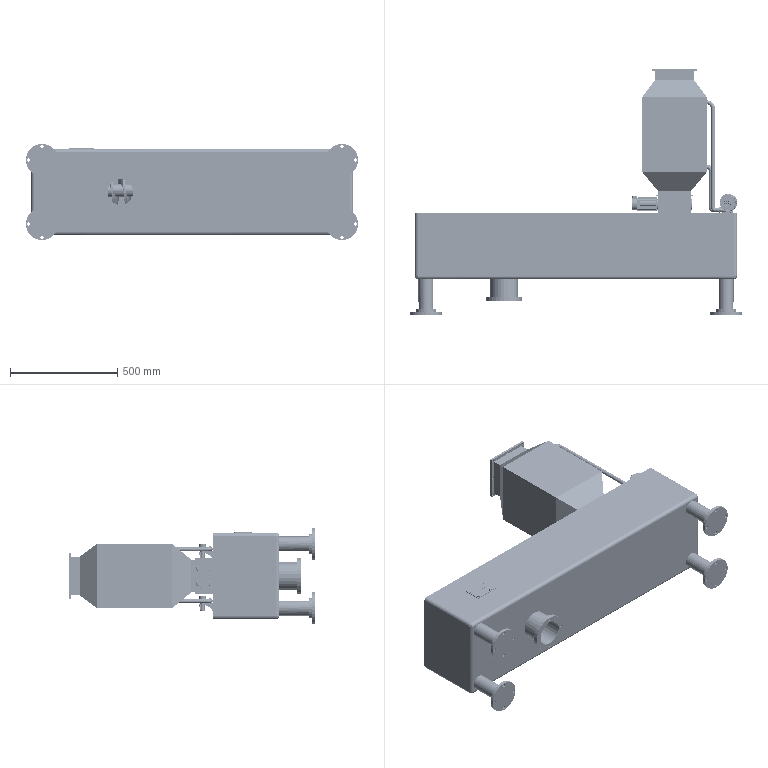Assembly | SolidWorks | mm | 45 component files | 49 solids | 6912 faces | box 1548.53 x 1145.2 x 448.53 mm | volume 120941884 mm3 | plane 3366 | cylinder 2732 | torus 522 | spline 126 | sphere 114 | cone 52 | commonest cylinder face diameters 0.75 x556 0.3 x432 15 x252 17 x208 6 x112 1.5 x64 10 x52 12.958 x45
Bill of materials:
90ST-M02430 | 2 |  | Motor-like body shaped as a long square-section housing. One end has a square mounting flange with four corner through-holes and a single cylindrical shaft. The other end has a short cylindrical rear cap with a small boxy protrusion on its side.
CrushingCutterBar | 2 |  | Solid straight cylindrical rod with a thin, slightly larger-diameter disc head at one end (pin- or rivet-like shape).
CrushingCutterDisc | 9 |  | Thick disc with a central round bore that has one rectangular keyway, and four curved, hook-shaped teeth evenly spaced around the rim and all curving the same way.
EndCover | 2 |  | Solid stepped disc: a larger-diameter disc joined coaxially to a thinner, smaller-diameter disc or boss on one face.
Fan | 2 |  | Assembly-like body that appears to be a centrifugal blower: a spiral (volute) housing with a tangential round outlet ending in a flange, a cylindrical housing on top with a perforated circular vent pattern, a finned cylindrical body and end cap below, a side box, and a plate bracket with mounting holes.
FeedBox | 1 |  | Rectangular box-shaped duct section with pyramidal tapers at both ends, each ending in a smaller rectangular neck with a bolted flange.
HeatPipe | 8 |  | Hollow round tube bent in one plane into a serpentine shape: six parallel straight runs joined by sharp, mitred-looking 180-degree returns, with both open ends on the same side.
PlateOne | 1 |  | Flat rectangular plate of uniform thickness with two round through-holes at diagonally opposite corners.
PlateTwo | 1 |  | Plain flat rectangular plate of uniform thickness with no visible holes or features.
Housing | 1 |  | Long rectangular box with lightly rounded edges. One long face carries four cylindrical stub pegs near its ends and a short round nozzle with a flange and small bolt holes. A small square opening is cut in the top face.
IMB3H56-90GeneralMotor[YS-561-4-B3] | 1 |  | Motor-like body shaped as a horizontal cylindrical housing. It has fins running along its length, bolt-down mounting feet with holes, and a rectangular box on top. A rounded cap covers one end. A small cylindrical shaft sticks out from the middle of the other end.
MotorEndCover | 2 |  | Stepped annular disc: a flat ring with a raised, smaller-diameter boss on one face and a central round bore with one rectangular keyway.
PipeOne | 1 |  | Hollow round tube with a long straight middle section and a short 90-degree bent leg at each end, the two legs pointing in opposite directions in one plane (Z or offset shape).
PipeTwo | 1 |  | Long, slender hollow round tube with small 90-degree bends at both ends turning in opposite directions in one plane (Z or offset shape). The close-up shows a chamfered end edge.
Screen | 1 |  | Thin rectangular plate with rounded corners. The top face has several low raised features, and a slightly smaller, thicker block sits under the plate.
SpiralConveyorRod | 1 |  | Straight cylindrical shaft with a continuous thin helical flight wrapped along its length. The shaft sticks out a short way past the flight at the end.
SupportFrame | 2 |  | Bent thin-plate bracket. A rectangular main face has two large round through-holes. A narrow side flange has three small holes, and there is a short return lip on the opposite edge.
SupportFrameA | 2 |  | Shallow U-shaped channel or cover made from thin plate: a flat rectangular top with two short downturned side flanges. One flange has three round holes.
SupportLeg | 4 |  | Flat circular disc with a large central through-bore and four smaller holes evenly spaced on a bolt circle. A raised hub of smaller diameter, concentric with the disc, sits on one face.
TopCover | 1 |  | Long, thin rectangular panel with rounded corners. It has one square through-cutout with small holes around its edge, and several thin rib or strip features running across the panel on one face.
Mates:
1. concentric | Housing-1 face at (-699.263, -180, 149.263) dir (0, 1, 0) r 35 | SupportLeg-2 face at (-699.263, -165, 149.263) dir (0, -1, 0) r 35
2. coincident | Housing-1 face at (-699.263, -180, 149.263) dir (0, -1, 0) | SupportLeg-2 face at (-699.263, -180, 149.263) dir (0, -1, 0)
3. coincident | Housing-1 face at (0, 0, 200) dir (0, 0, 1) | TopCover-1 face at (-734.95, 285, 200) dir (0, 0, 1)
4. coincident | Housing-1 face at (-750, 0, 0) dir (-1, 0, 0) | TopCover-1 face at (-750, 285, -184.95) dir (-1, 0, 0)
5. coincident | Housing-1 face at (-750, 285, -200) dir (0, 1, 0) | TopCover-1 face at (734.95, 285, -184.95) dir (0, -1, 0)
6. concentric | Housing-1 face at (-454, 142.868, 6.9) dir (1, 0, 0) r 30 | SpiralConveyorRod-2 face at (-407, 142.868, 6.9) dir (1, 0, 0) r 30
7. coincident | TopCover-1 face at (734.95, 295, -184.95) dir (0, 1, 0) | SupportFrame-1 face at (384.19, 295, 85) dir (0, -1, 0)
8. coincident | TopCover-1 face at (384.29, 72.868, -75) dir (1, 0, 0) | SupportFrame-1 face at (384.29, 295.1, 85) dir (1, 0, 0)
9. distance | SupportFrame-1 face at (384.19, 311.439, -85) dir (0, 0, -1) | TopCover-1 face at (384.29, 72.868, -75) dir (0, 0, 1)
10. coincident | TopCover-1 face at (534.29, 72.868, -75) dir (-1, 0, 0) | SupportFrame-2 face at (534.29, 295.1, -85) dir (-1, 0, 0)
11. coincident | TopCover-1 face at (734.95, 295, -184.95) dir (0, 1, 0) | SupportFrame-2 face at (534.39, 295, -85) dir (0, -1, 0)
12. distance | SupportFrame-2 face at (534.39, 295.1, -85) dir (0, 0, -1) | TopCover-1 face at (384.29, 72.868, -75) dir (0, 0, 1)
13. coincident | TopCover-1 face at (734.95, 295, -184.95) dir (0, 1, 0) | SupportFrameA-2 face at (384.29, 295, -75.5) dir (0, -1, 0)
14. coincident | TopCover-1 face at (384.29, 72.868, -75) dir (0, 0, 1) | SupportFrameA-2 face at (384.29, 295.5, -75) dir (0, 0, 1)
15. coincident | SupportFrameA-2 face at (534.29, 374.7, -75.5) dir (1, 0, 0) | SupportFrame-2 face at (534.29, 295.1, -85) dir (-1, 0, 0)
16. coincident | TopCover-1 face at (734.95, 295, -184.95) dir (0, 1, 0) | SupportFrameA-3 face at (534.29, 295, 75.5) dir (0, -1, 0)
17. coincident | TopCover-1 face at (384.29, 72.868, 75) dir (0, 0, -1) | SupportFrameA-3 face at (534.29, 295.5, 75) dir (0, 0, -1)
18. coincident | SupportFrame-1 face at (384.29, 295.1, 85) dir (1, 0, 0) | SupportFrameA-3 face at (384.29, 295.5, 75.5) dir (-1, 0, 0)
19. concentric | SpiralConveyorRod-2 edge at (-407, 142.868, 6.9) dir (1, 0, 0) r 30 | IMB3H56-90GeneralMotor[YS-561-4-B3]-2 face at (-410, 142.868, 6.9) dir (-1, 0, 0) r 4.5
20. coincident | Housing-1 face at (-410, 0, 0) dir (-1, 0, 0) | IMB3H56-90GeneralMotor[YS-561-4-B3]-2 face at (-410, 117.868, 6.9) dir (1, 0, 0)
21. concentric | SupportFrame-1 edge at (384.19, 335.1, 35) dir (-1, 0, 0) r 20 | 60-90SeriesServoMotor[60ST-M00630]-1 face at (403.19, 335.1, 35) dir (1, 0, 0) r 6
22. concentric | SupportFrame-1 edge at (384.19, 335.1, -35) dir (-1, 0, 0) r 20 | 60-90SeriesServoMotor[60ST-M00630]-2 face at (403.19, 335.1, -35) dir (1, 0, 0) r 6
23. parallel | TopCover-1 face at (734.95, 295, -184.95) dir (0, 1, 0) | 60-90SeriesServoMotor[60ST-M00630]-1 face at (370.94, 367.35, 62.375) dir (0, 1, 0)
24. parallel | TopCover-1 face at (734.95, 295, -184.95) dir (0, 1, 0) | 60-90SeriesServoMotor[60ST-M00630]-2 face at (370.94, 367.35, -7.625) dir (0, 1, 0)
25. concentric | SupportFrame-1 edge at (384.19, 335.1, 35) dir (-1, 0, 0) r 20 | MotorEndCover-1 face at (386.19, 335.1, 35) dir (1, 0, 0) r 8
26. concentric | SupportFrame-1 edge at (384.19, 335.1, -35) dir (-1, 0, 0) r 20 | MotorEndCover-2 edge at (379.19, 335.1, -35) dir (1, 0, 0) r 8
27. coincident | SupportFrame-1 face at (384.19, 295.1, 85) dir (-1, 0, 0) | MotorEndCover-2 face at (384.19, 335.1, -35) dir (1, 0, 0)
28. coincident | 60-90SeriesServoMotor[60ST-M00630]-1 face at (379.19, 335.1, 35) dir (1, 0, 0) | MotorEndCover-1 face at (379.19, 335.1, 35) dir (-1, 0, 0)
29. coincident | 60-90SeriesServoMotor[60ST-M00630]-2 face at (379.19, 335.1, -35) dir (1, 0, 0) | MotorEndCover-2 face at (379.19, 335.1, -35) dir (-1, 0, 0)
30. concentric | 60-90SeriesServoMotor[60ST-M00630]-2 face at (403.19, 335.1, -35) dir (1, 0, 0) r 6 | CrushingCutterBar-1 face at (529.19, 335.1, -35) dir (-1, 0, 0) r 8
31. coincident | MotorEndCover-2 face at (386.19, 335.1, -35) dir (1, 0, 0) | CrushingCutterBar-1 face at (386.19, 335.1, -35) dir (-1, 0, 0)
32. concentric | SupportFrame-2 edge at (534.39, 335.1, -35) dir (1, 0, 0) r 20 | EndCover-1 edge at (529.39, 335.1, -35) dir (-1, 0, 0) r 14.92
33. coincident | SupportFrame-2 face at (534.39, 295.1, -85) dir (1, 0, 0) | EndCover-1 face at (534.39, 335.1, -35) dir (-1, 0, 0)
34. concentric | 60-90SeriesServoMotor[60ST-M00630]-1 edge at (402.695, 335.1, 35) dir (-1, 0, 0) r 6 | CrushingCutterBar-2 edge at (386.19, 335.1, 35) dir (1, 0, 0) r 8
35. parallel | 60-90SeriesServoMotor[60ST-M00630]-2 face at (384.065, 342.6, -35) dir (0, 1, 0) | CrushingCutterBar-1 face at (529.19, 349.808, -32.501) dir (0, 1, 0)
36. parallel | 60-90SeriesServoMotor[60ST-M00630]-1 face at (384.065, 342.6, 35) dir (0, 1, 0) | CrushingCutterBar-2 face at (529.19, 349.808, 37.499) dir (0, 1, 0)
37. coincident | MotorEndCover-1 face at (386.19, 335.1, 35) dir (1, 0, 0) | CrushingCutterBar-2 face at (386.19, 335.1, 35) dir (-1, 0, 0)
38. concentric | CrushingCutterBar-2 edge at (531.19, 335.1, 35) dir (1, 0, 0) r 14.919 | EndCover-2 edge at (529.39, 335.1, 35) dir (-1, 0, 0) r 14.92
39. coincident | SupportFrame-2 face at (534.39, 295.1, -85) dir (1, 0, 0) | EndCover-2 face at (534.39, 335.1, 35) dir (-1, 0, 0)
40. concentric | CrushingCutterBar-1 face at (529.19, 335.1, -35) dir (-1, 0, 0) r 12.5 | CrushingCutterDisc-1 face at (386.19, 335.1, -35) dir (1, 0, 0) r 12.5
41. coincident | CrushingCutterBar-1 face at (529.19, 347.348, -32.501) dir (0, 0, 1) | CrushingCutterDisc-1 face at (386.19, 347.348, -32.501) dir (0, 0, -1)
42. coincident | MotorEndCover-2 face at (386.19, 335.1, -35) dir (1, 0, 0) | CrushingCutterDisc-1 face at (386.19, 341.527, -19.472) dir (-1, 0, 0)
43. concentric | CrushingCutterBar-2 face at (529.19, 335.1, 35) dir (-1, 0, 0) r 12.5 | CrushingCutterDisc-6 face at (401.909, 335.1, 35) dir (1, 0, 0) r 12.5
44. coincident | CrushingCutterBar-2 face at (529.19, 347.348, 37.499) dir (0, 0, 1) | CrushingCutterDisc-6 face at (401.909, 347.348, 37.499) dir (0, 0, -1)
45. coincident | Housing-1 face at (-565, 195, 200) dir (1, 0, 0) | Screen-1 face at (-565, 118.296, 200) dir (-1, 0, 0)
46. coincident | Housing-1 face at (-565, 195, 200) dir (0, -1, 0) | Screen-1 face at (-575.173, 195, 203) dir (0, 1, 0)
47. coincident | Housing-1 face at (0, 0, 200) dir (0, 0, 1) | Screen-1 face at (-565, 118.296, 200) dir (0, 0, -1)
48. coincident | SupportFrame-1 face at (384.19, 375.2, 85) dir (0, 1, 0) | FeedBox-1 face at (458.89, 375.2, 0) dir (0, -1, 0)
49. concentric | SupportFrame-2 face at (539.39, 375.2, -55) dir (0, -1, 0) r 3 | FeedBox-1 face at (539.39, 377.2, -55) dir (0, -1, 0) r 3
50. parallel | SupportFrameA-3 face at (534.29, 374.7, 85.5) dir (0, 0, 1) | FeedBox-1 face at (458.89, 377.2, 85) dir (0, 0, 1)
51. parallel | TopCover-1 face at (750, 285, -184.95) dir (1, 0, 0) | Fan-1 face at (732.155, 383.773, -84.437) dir (1, 0, 0)
52. coincident | TopCover-1 face at (734.95, 295, -184.95) dir (0, 1, 0) | Fan-1 face at (707.155, 295, -117.25) dir (0, -1, 0)
53. concentric | PipeOne-1 face at (638.89, 309.375, -117.25) dir (1, 0, 0) r 7.5 | Fan-1 face at (667.28, 309.375, -117.25) dir (-1, 0, 0) r 87.266
54. parallel | TopCover-1 face at (750, 285, -184.95) dir (1, 0, 0) | Fan-2 face at (732.155, 383.773, 157.813) dir (1, 0, 0)
55. coincident | TopCover-1 face at (734.95, 295, -184.95) dir (0, 1, 0) | Fan-2 face at (707.155, 295, 125) dir (0, -1, 0)
56. coincident | Fan-1 face at (732.155, 383.773, -84.437) dir (1, 0, 0) | Fan-2 face at (732.155, 383.773, 157.813) dir (1, 0, 0)
57. concentric | FeedBox-1 edge at (606.39, 810.2, 125) dir (1, 0, 0) r 9.4 | PipeTwo-1 edge at (602.005, 810.2, 125) dir (-1, 0, 0) r 7.5
58. concentric | PipeTwo-1 edge at (608.89, 810.2, 125) dir (-1, 0, 0) r 9.385 | HeatExchangePlate-1/HeatPipe-1 edge at (586.39, 810.2, 125) dir (1, 0, 0) r 8.5
59. coincident | FeedBox-1 face at (606.39, 835.2, -147.5) dir (-1, 0, 0) | HeatExchangePlate-1/PlateOne-1 face at (606.39, 1046.117, 185.761) dir (1, 0, 0)
60. coincident | SupportFrame-1 face at (384.19, 295.1, 85) dir (-1, 0, 0) | MotorEndCover-1 face at (384.19, 335.1, 35) dir (1, 0, 0)
61. coincident | PlateOne-1 face at (-28.489, 120.787, 1010) dir (0, 0, 1) | HeatPipe-1 face at (-89.25, -115.13, 1010) dir (0, 0, -1)
62. concentric | PlateOne-1 edge at (-89.25, -115.13, 1010) dir (0, 0, 1) r 8.5 | HeatPipe-1 edge at (-89.25, -115.13, 1010) dir (0, 0, -1) r 8.5
63. coincident | PlateOne-1 face at (-79.5, -440.12, 1010) dir (0, -1, 0) | PlateTwo-1 edge at (-346.852, -440.12, 1285) dir (1, 0, 0)
64. parallel | PlateOne-1 face at (-341.177, -105.38, 1010) dir (0, 1, 0) | PlateTwo-1 face at (-346.852, -105.38, 1285) dir (0, 1, 0)
65. coincident | PlateOne-1 face at (-346.852, -440.12, 1010) dir (-1, 0, 0) | PlateTwo-1 face at (-346.852, -105.38, 1285) dir (-1, 0, 0)